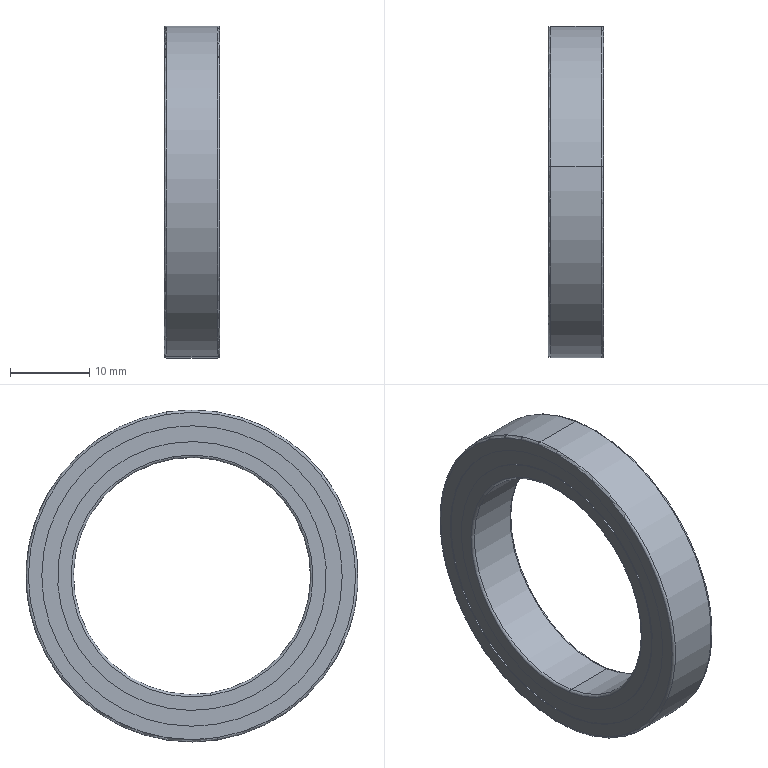Component | SolidWorks | DeepGrooveBallBearing6204-2 | 34 solids | 184 faces | volume 3590 mm3 | sphere 124 | cylinder 24 | torus 14 | cone 12 | plane 10 | commonest cylinder face diameters 38 x6 34 x6 38.6 x4 33.4 x4 42 x2 30 x2